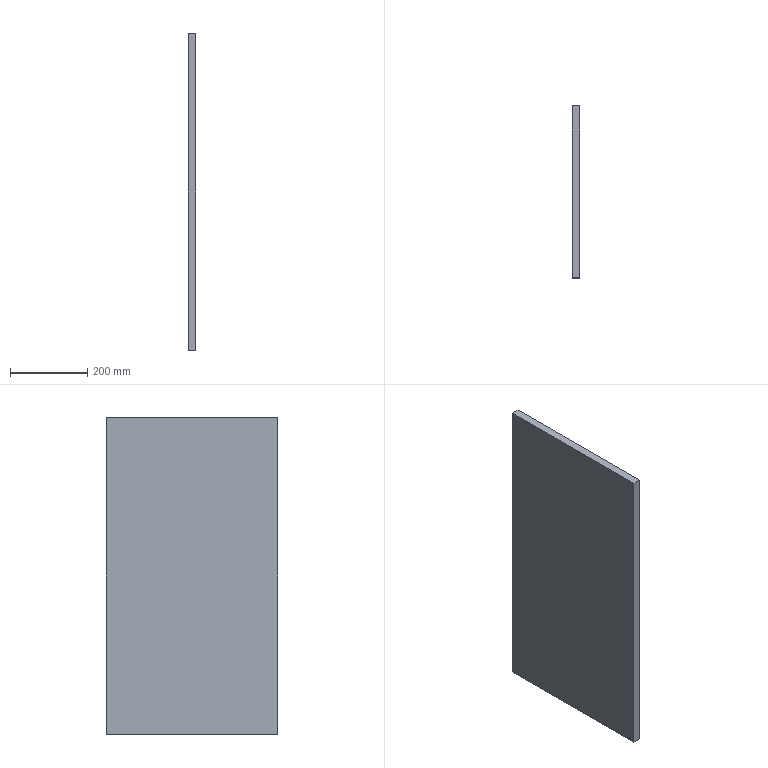Component | SolidWorks | SupportPlate-1 | 1 solid | 6 faces | box 20 x 444 x 820 mm | volume 7281600 mm3 | plane 6
build123d program:
from build123d import *

# Parameters (mm, degrees)
SKETCH1_W           = 820
SKETCH1_H           = 444
BOSS_EXTRUDE1_DEPTH = 20


with BuildPart() as part:
    # Sketch1 → Boss-Extrude1 (new body)
    with BuildSketch(Plane(origin=(0, 0, 0), x_dir=(0, 0, -1), z_dir=(1, 0, 0))):
        Rectangle(SKETCH1_W, SKETCH1_H)
    extrude(amount=BOSS_EXTRUDE1_DEPTH)


solid = part.part

# Placed as in the assembly
solid = solid.moved(Location((-200.267, 15.31, 90), (0, 0, 0)))
STEP:
#1=COLOUR_RGB('',0.7922,0.8196,0.9333);
#2=FILL_AREA_STYLE_COLOUR('',#1);
#3=FILL_AREA_STYLE('',(#2));
#4=SURFACE_STYLE_FILL_AREA(#3);
#5=SURFACE_SIDE_STYLE('',(#4));
#6=SURFACE_STYLE_USAGE(.BOTH.,#5);
#7=PRESENTATION_STYLE_ASSIGNMENT((#6));
#8=CARTESIAN_POINT('',(-7.885,9.343,19.685));
#9=VERTEX_POINT('',#8);
#10=CARTESIAN_POINT('',(-7.885,-8.137,19.685));
#11=VERTEX_POINT('',#10);
#12=CARTESIAN_POINT('',(-7.885,9.343,19.685));
#13=DIRECTION('',(0.,-1.,-0.));
#14=VECTOR('',#13,39.37);
#15=LINE('',#12,#14);
#16=EDGE_CURVE('',#9,#11,#15,.T.);
#17=ORIENTED_EDGE('',*,*,#16,.T.);
#18=CARTESIAN_POINT('',(-7.097,-8.137,19.685));
#19=VERTEX_POINT('',#18);
#20=CARTESIAN_POINT('',(-7.097,-8.137,19.685));
#21=DIRECTION('',(-1.,0.,0.));
#22=VECTOR('',#21,39.37);
#23=LINE('',#20,#22);
#24=EDGE_CURVE('',#19,#11,#23,.T.);
#25=ORIENTED_EDGE('',*,*,#24,.F.);
#26=CARTESIAN_POINT('',(-7.097,9.343,19.685));
#27=VERTEX_POINT('',#26);
#28=CARTESIAN_POINT('',(-7.097,9.343,19.685));
#29=DIRECTION('',(0.,-1.,-0.));
#30=VECTOR('',#29,39.37);
#31=LINE('',#28,#30);
#32=EDGE_CURVE('',#27,#19,#31,.T.);
#33=ORIENTED_EDGE('',*,*,#32,.F.);
#34=CARTESIAN_POINT('',(-7.097,9.343,19.685));
#35=DIRECTION('',(-1.,0.,0.));
#36=VECTOR('',#35,39.37);
#37=LINE('',#34,#36);
#38=EDGE_CURVE('',#27,#9,#37,.T.);
#39=ORIENTED_EDGE('',*,*,#38,.T.);
#40=EDGE_LOOP('',(#17,#25,#33,#39));
#41=FACE_OUTER_BOUND('',#40,.T.);
#42=CARTESIAN_POINT('',(-7.097,9.343,19.685));
#43=DIRECTION('',(0.,0.,-1.));
#44=DIRECTION('',(0.,1.,0.));
#45=AXIS2_PLACEMENT_3D('',#42,#43,#44);
#46=PLANE('',#45);
#47=ADVANCED_FACE('',(#41),#46,.F.);
#48=CARTESIAN_POINT('',(-7.885,-8.137,-12.598));
#49=VERTEX_POINT('',#48);
#50=CARTESIAN_POINT('',(-7.885,-8.137,-12.598));
#51=DIRECTION('',(0.,0.,-1.));
#52=VECTOR('',#51,39.37);
#53=LINE('',#50,#52);
#54=EDGE_CURVE('',#11,#49,#53,.T.);
#55=ORIENTED_EDGE('',*,*,#54,.T.);
#56=CARTESIAN_POINT('',(-7.097,-8.137,-12.598));
#57=VERTEX_POINT('',#56);
#58=CARTESIAN_POINT('',(-7.097,-8.137,-12.598));
#59=DIRECTION('',(-1.,0.,0.));
#60=VECTOR('',#59,39.37);
#61=LINE('',#58,#60);
#62=EDGE_CURVE('',#57,#49,#61,.T.);
#63=ORIENTED_EDGE('',*,*,#62,.F.);
#64=CARTESIAN_POINT('',(-7.097,-8.137,-12.598));
#65=DIRECTION('',(0.,0.,-1.));
#66=VECTOR('',#65,39.37);
#67=LINE('',#64,#66);
#68=EDGE_CURVE('',#19,#57,#67,.T.);
#69=ORIENTED_EDGE('',*,*,#68,.F.);
#70=ORIENTED_EDGE('',*,*,#24,.T.);
#71=EDGE_LOOP('',(#55,#63,#69,#70));
#72=FACE_OUTER_BOUND('',#71,.T.);
#73=CARTESIAN_POINT('',(-7.097,-8.137,-12.598));
#74=DIRECTION('',(0.,1.,0.));
#75=DIRECTION('',(0.,-0.,1.));
#76=AXIS2_PLACEMENT_3D('',#73,#74,#75);
#77=PLANE('',#76);
#78=ADVANCED_FACE('',(#72),#77,.F.);
#79=CARTESIAN_POINT('',(-7.885,9.343,-12.598));
#80=VERTEX_POINT('',#79);
#81=CARTESIAN_POINT('',(-7.885,9.343,-12.598));
#82=DIRECTION('',(0.,1.,0.));
#83=VECTOR('',#82,39.37);
#84=LINE('',#81,#83);
#85=EDGE_CURVE('',#49,#80,#84,.T.);
#86=ORIENTED_EDGE('',*,*,#85,.T.);
#87=CARTESIAN_POINT('',(-7.097,9.343,-12.598));
#88=VERTEX_POINT('',#87);
#89=CARTESIAN_POINT('',(-7.097,9.343,-12.598));
#90=DIRECTION('',(-1.,0.,0.));
#91=VECTOR('',#90,39.37);
#92=LINE('',#89,#91);
#93=EDGE_CURVE('',#88,#80,#92,.T.);
#94=ORIENTED_EDGE('',*,*,#93,.F.);
#95=CARTESIAN_POINT('',(-7.097,9.343,-12.598));
#96=DIRECTION('',(0.,1.,0.));
#97=VECTOR('',#96,39.37);
#98=LINE('',#95,#97);
#99=EDGE_CURVE('',#57,#88,#98,.T.);
#100=ORIENTED_EDGE('',*,*,#99,.F.);
#101=ORIENTED_EDGE('',*,*,#62,.T.);
#102=EDGE_LOOP('',(#86,#94,#100,#101));
#103=FACE_OUTER_BOUND('',#102,.T.);
#104=CARTESIAN_POINT('',(-7.097,9.343,-12.598));
#105=DIRECTION('',(0.,-0.,1.));
#106=DIRECTION('',(0.,-1.,-0.));
#107=AXIS2_PLACEMENT_3D('',#104,#105,#106);
#108=PLANE('',#107);
#109=ADVANCED_FACE('',(#103),#108,.F.);
#110=CARTESIAN_POINT('',(-7.885,9.343,-12.598));
#111=DIRECTION('',(0.,-0.,1.));
#112=VECTOR('',#111,39.37);
#113=LINE('',#110,#112);
#114=EDGE_CURVE('',#80,#9,#113,.T.);
#115=ORIENTED_EDGE('',*,*,#114,.T.);
#116=ORIENTED_EDGE('',*,*,#38,.F.);
#117=CARTESIAN_POINT('',(-7.097,9.343,-12.598));
#118=DIRECTION('',(0.,-0.,1.));
#119=VECTOR('',#118,39.37);
#120=LINE('',#117,#119);
#121=EDGE_CURVE('',#88,#27,#120,.T.);
#122=ORIENTED_EDGE('',*,*,#121,.F.);
#123=ORIENTED_EDGE('',*,*,#93,.T.);
#124=EDGE_LOOP('',(#115,#116,#122,#123));
#125=FACE_OUTER_BOUND('',#124,.T.);
#126=CARTESIAN_POINT('',(-7.097,9.343,-12.598));
#127=DIRECTION('',(0.,-1.,-0.));
#128=DIRECTION('',(0.,0.,-1.));
#129=AXIS2_PLACEMENT_3D('',#126,#127,#128);
#130=PLANE('',#129);
#131=ADVANCED_FACE('',(#125),#130,.F.);
#132=ORIENTED_EDGE('',*,*,#32,.T.);
#133=ORIENTED_EDGE('',*,*,#68,.T.);
#134=ORIENTED_EDGE('',*,*,#99,.T.);
#135=ORIENTED_EDGE('',*,*,#121,.T.);
#136=EDGE_LOOP('',(#132,#133,#134,#135));
#137=FACE_OUTER_BOUND('',#136,.T.);
#138=CARTESIAN_POINT('',(-7.097,0.6028,3.543));
#139=DIRECTION('',(-1.,0.,0.));
#140=DIRECTION('',(0.,0.,1.));
#141=AXIS2_PLACEMENT_3D('',#138,#139,#140);
#142=PLANE('',#141);
#143=ADVANCED_FACE('',(#137),#142,.F.);
#144=ORIENTED_EDGE('',*,*,#16,.F.);
#145=ORIENTED_EDGE('',*,*,#114,.F.);
#146=ORIENTED_EDGE('',*,*,#85,.F.);
#147=ORIENTED_EDGE('',*,*,#54,.F.);
#148=EDGE_LOOP('',(#144,#145,#146,#147));
#149=FACE_OUTER_BOUND('',#148,.T.);
#150=CARTESIAN_POINT('',(-7.885,0.6028,3.543));
#151=DIRECTION('',(-1.,0.,0.));
#152=DIRECTION('',(0.,0.,1.));
#153=AXIS2_PLACEMENT_3D('',#150,#151,#152);
#154=PLANE('',#153);
#155=ADVANCED_FACE('',(#149),#154,.T.);
#156=CLOSED_SHELL('',(#47,#78,#109,#131,#143,#155));
#157=MANIFOLD_SOLID_BREP('',#156);
#158=STYLED_ITEM('',(#7),#157);
#159=PRESENTATION_LAYER_ASSIGNMENT('','',(#158));
#160=(LENGTH_UNIT()NAMED_UNIT(*)SI_UNIT($,.METRE.));
#161=LENGTH_MEASURE_WITH_UNIT(LENGTH_MEASURE(0.0254),#160);
#162=DIMENSIONAL_EXPONENTS(1.,0.,0.,0.,0.,0.,0.);
#163=(CONVERSION_BASED_UNIT('',#161)LENGTH_UNIT()NAMED_UNIT(#162));
#164=UNCERTAINTY_MEASURE_WITH_UNIT(LENGTH_MEASURE(0.00001),#163,'','');
#165=(NAMED_UNIT(*)PLANE_ANGLE_UNIT()SI_UNIT($,.RADIAN.));
#166=(NAMED_UNIT(*)SI_UNIT($,.STERADIAN.)SOLID_ANGLE_UNIT());
#167=(GEOMETRIC_REPRESENTATION_CONTEXT(3)GLOBAL_UNCERTAINTY_ASSIGNED_CONTEXT((#164))GLOBAL_UNIT_ASSIGNED_CONTEXT((#163,#165,#166))REPRESENTATION_CONTEXT('',''));
#168=MECHANICAL_DESIGN_GEOMETRIC_PRESENTATION_REPRESENTATION('',(#158),#167);
#169=CARTESIAN_POINT('',(0.,0.,0.));
#170=DIRECTION('',(0.,0.,1.));
#171=DIRECTION('',(1.,0.,0.));
#172=AXIS2_PLACEMENT_3D('',#169,#170,#171);
#173=(LENGTH_UNIT()NAMED_UNIT(*)SI_UNIT($,.METRE.));
#174=LENGTH_MEASURE_WITH_UNIT(LENGTH_MEASURE(0.0254),#173);
#175=DIMENSIONAL_EXPONENTS(1.,0.,0.,0.,0.,0.,0.);
#176=(CONVERSION_BASED_UNIT('',#174)LENGTH_UNIT()NAMED_UNIT(#175));
#177=UNCERTAINTY_MEASURE_WITH_UNIT(LENGTH_MEASURE(0.00001),#176,'','');
#178=(NAMED_UNIT(*)PLANE_ANGLE_UNIT()SI_UNIT($,.RADIAN.));
#179=(NAMED_UNIT(*)SI_UNIT($,.STERADIAN.)SOLID_ANGLE_UNIT());
#180=(GEOMETRIC_REPRESENTATION_CONTEXT(3)GLOBAL_UNCERTAINTY_ASSIGNED_CONTEXT((#177))GLOBAL_UNIT_ASSIGNED_CONTEXT((#176,#178,#179))REPRESENTATION_CONTEXT('',''));
#181=ADVANCED_BREP_SHAPE_REPRESENTATION('',(#157,#172),#180);